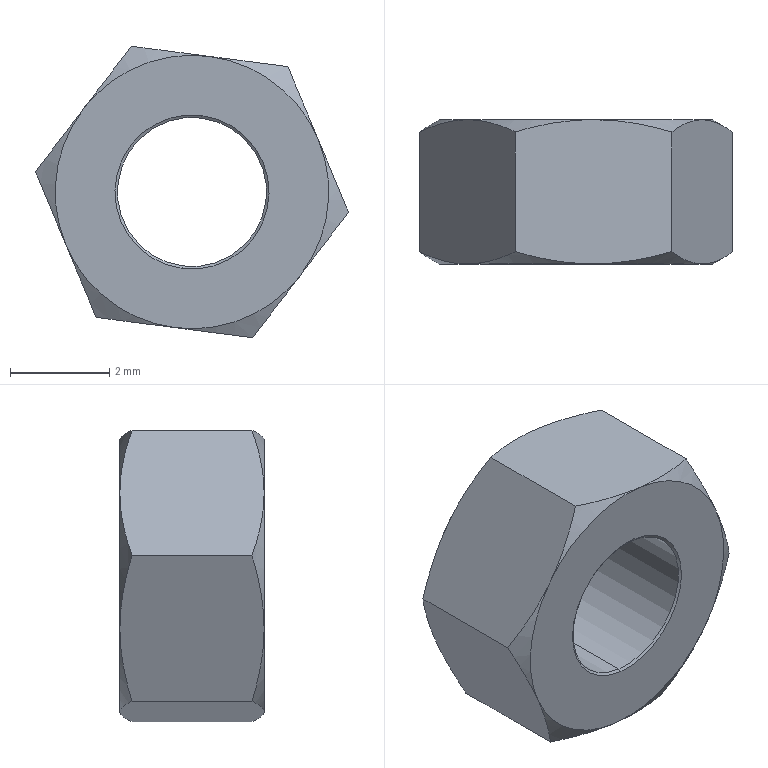Component | SolidWorks | hex nut style 2_am_pkg-1 | 1 solid | 28 faces | box 6.3 x 2.9 x 5.86 mm | volume 55 mm3 | cone 16 | plane 8 | cylinder 4 | commonest cylinder face diameters 3.1 x2 3 x2
STEP:
#1=COLOUR_RGB('',0.7922,0.8196,0.9333);
#2=FILL_AREA_STYLE_COLOUR('',#1);
#3=FILL_AREA_STYLE('',(#2));
#4=SURFACE_STYLE_FILL_AREA(#3);
#5=SURFACE_SIDE_STYLE('',(#4));
#6=SURFACE_STYLE_USAGE(.BOTH.,#5);
#7=PRESENTATION_STYLE_ASSIGNMENT((#6));
#8=CARTESIAN_POINT('',(-0.8987,-0.,1.164));
#9=VERTEX_POINT('',#8);
#10=CARTESIAN_POINT('',(-0.883,-0.,1.285));
#11=VERTEX_POINT('',#10);
#12=CARTESIAN_POINT('',(-0.8908,-0.,1.225));
#13=DIRECTION('',(0.,-1.,0.));
#14=DIRECTION('',(-0.1287,-0.,-0.9917));
#15=AXIS2_PLACEMENT_3D('',#12,#13,#14);
#16=CIRCLE('',#15,0.06102);
#17=EDGE_CURVE('',#9,#11,#16,.T.);
#18=ORIENTED_EDGE('',*,*,#17,.F.);
#19=CARTESIAN_POINT('',(-0.8987,-0.001,1.164));
#20=VERTEX_POINT('',#19);
#21=CARTESIAN_POINT('',(-0.8987,0.8716,1.164));
#22=DIRECTION('',(0.,-1.,0.));
#23=VECTOR('',#22,39.37);
#24=LINE('',#21,#23);
#25=EDGE_CURVE('',#9,#20,#24,.T.);
#26=ORIENTED_EDGE('',*,*,#25,.T.);
#27=CARTESIAN_POINT('',(-0.883,-0.001,1.285));
#28=VERTEX_POINT('',#27);
#29=CARTESIAN_POINT('',(-0.8908,-0.001,1.225));
#30=DIRECTION('',(0.,-1.,0.));
#31=DIRECTION('',(0.1287,0.,0.9917));
#32=AXIS2_PLACEMENT_3D('',#29,#30,#31);
#33=CIRCLE('',#32,0.06102);
#34=EDGE_CURVE('',#20,#28,#33,.T.);
#35=ORIENTED_EDGE('',*,*,#34,.T.);
#36=CARTESIAN_POINT('',(-0.883,0.8716,1.285));
#37=DIRECTION('',(0.,-1.,0.));
#38=VECTOR('',#37,39.37);
#39=LINE('',#36,#38);
#40=EDGE_CURVE('',#11,#28,#39,.T.);
#41=ORIENTED_EDGE('',*,*,#40,.F.);
#42=EDGE_LOOP('',(#18,#26,#35,#41));
#43=FACE_OUTER_BOUND('',#42,.T.);
#44=CARTESIAN_POINT('',(-0.8908,0.8716,1.225));
#45=DIRECTION('',(0.,-1.,0.));
#46=DIRECTION('',(0.1287,0.,0.9917));
#47=AXIS2_PLACEMENT_3D('',#44,#45,#46);
#48=CYLINDRICAL_SURFACE('',#47,0.06102);
#49=ADVANCED_FACE('',(#43),#48,.F.);
#50=CARTESIAN_POINT('',(-0.8984,-0.002378,1.166));
#51=VERTEX_POINT('',#50);
#52=CARTESIAN_POINT('',(-0.8832,-0.002378,1.283));
#53=VERTEX_POINT('',#52);
#54=CARTESIAN_POINT('',(-0.8908,-0.002378,1.225));
#55=DIRECTION('',(0.,-1.,0.));
#56=DIRECTION('',(-0.1287,-0.,-0.9917));
#57=AXIS2_PLACEMENT_3D('',#54,#55,#56);
#58=CIRCLE('',#57,0.05906);
#59=EDGE_CURVE('',#51,#53,#58,.T.);
#60=ORIENTED_EDGE('',*,*,#59,.T.);
#61=CARTESIAN_POINT('',(-0.883,-0.001,1.285));
#62=DIRECTION('',(0.1054,0.5736,0.8123));
#63=VECTOR('',#62,39.37);
#64=LINE('',#61,#63);
#65=EDGE_CURVE('',#53,#28,#64,.T.);
#66=ORIENTED_EDGE('',*,*,#65,.T.);
#67=ORIENTED_EDGE('',*,*,#34,.F.);
#68=CARTESIAN_POINT('',(-0.8987,-0.001,1.164));
#69=DIRECTION('',(-0.1054,0.5736,-0.8123));
#70=VECTOR('',#69,39.37);
#71=LINE('',#68,#70);
#72=EDGE_CURVE('',#51,#20,#71,.T.);
#73=ORIENTED_EDGE('',*,*,#72,.F.);
#74=EDGE_LOOP('',(#60,#66,#67,#73));
#75=FACE_OUTER_BOUND('',#74,.T.);
#76=CARTESIAN_POINT('',(-0.8908,-0.001,1.225));
#77=DIRECTION('',(-0.,1.,-0.));
#78=DIRECTION('',(-0.1287,-0.,-0.9917));
#79=AXIS2_PLACEMENT_3D('',#76,#77,#78);
#80=CONICAL_SURFACE('',#79,0.06102,0.9599);
#81=ADVANCED_FACE('',(#75),#80,.F.);
#82=CARTESIAN_POINT('',(-0.8832,-0.1128,1.283));
#83=VERTEX_POINT('',#82);
#84=CARTESIAN_POINT('',(-0.8984,-0.1128,1.166));
#85=VERTEX_POINT('',#84);
#86=CARTESIAN_POINT('',(-0.8908,-0.1128,1.225));
#87=DIRECTION('',(-0.,1.,-0.));
#88=DIRECTION('',(0.1287,0.,0.9917));
#89=AXIS2_PLACEMENT_3D('',#86,#87,#88);
#90=CIRCLE('',#89,0.05906);
#91=EDGE_CURVE('',#83,#85,#90,.T.);
#92=ORIENTED_EDGE('',*,*,#91,.T.);
#93=CARTESIAN_POINT('',(-0.8987,-0.1142,1.164));
#94=VERTEX_POINT('',#93);
#95=CARTESIAN_POINT('',(-0.8984,-0.1127,1.167));
#96=DIRECTION('',(-0.1054,-0.5736,-0.8123));
#97=VECTOR('',#96,39.37);
#98=LINE('',#95,#97);
#99=EDGE_CURVE('',#85,#94,#98,.T.);
#100=ORIENTED_EDGE('',*,*,#99,.T.);
#101=CARTESIAN_POINT('',(-0.883,-0.1142,1.285));
#102=VERTEX_POINT('',#101);
#103=CARTESIAN_POINT('',(-0.8908,-0.1142,1.225));
#104=DIRECTION('',(0.,-1.,0.));
#105=DIRECTION('',(0.1287,0.,0.9917));
#106=AXIS2_PLACEMENT_3D('',#103,#104,#105);
#107=CIRCLE('',#106,0.06102);
#108=EDGE_CURVE('',#94,#102,#107,.T.);
#109=ORIENTED_EDGE('',*,*,#108,.T.);
#110=CARTESIAN_POINT('',(-0.8833,-0.1127,1.283));
#111=DIRECTION('',(0.1054,-0.5736,0.8123));
#112=VECTOR('',#111,39.37);
#113=LINE('',#110,#112);
#114=EDGE_CURVE('',#83,#102,#113,.T.);
#115=ORIENTED_EDGE('',*,*,#114,.F.);
#116=EDGE_LOOP('',(#92,#100,#109,#115));
#117=FACE_OUTER_BOUND('',#116,.T.);
#118=CARTESIAN_POINT('',(-0.8908,-0.1127,1.225));
#119=DIRECTION('',(0.,-1.,0.));
#120=DIRECTION('',(0.1287,0.,0.9917));
#121=AXIS2_PLACEMENT_3D('',#118,#119,#120);
#122=CONICAL_SURFACE('',#121,0.05886,0.9599);
#123=ADVANCED_FACE('',(#117),#122,.F.);
#124=ORIENTED_EDGE('',*,*,#59,.F.);
#125=CARTESIAN_POINT('',(-0.8984,-0.,1.166));
#126=DIRECTION('',(0.,-1.,0.));
#127=VECTOR('',#126,39.37);
#128=LINE('',#125,#127);
#129=EDGE_CURVE('',#51,#85,#128,.T.);
#130=ORIENTED_EDGE('',*,*,#129,.T.);
#131=ORIENTED_EDGE('',*,*,#91,.F.);
#132=CARTESIAN_POINT('',(-0.8832,-0.,1.283));
#133=DIRECTION('',(0.,-1.,0.));
#134=VECTOR('',#133,39.37);
#135=LINE('',#132,#134);
#136=EDGE_CURVE('',#53,#83,#135,.T.);
#137=ORIENTED_EDGE('',*,*,#136,.F.);
#138=EDGE_LOOP('',(#124,#130,#131,#137));
#139=FACE_OUTER_BOUND('',#138,.T.);
#140=CARTESIAN_POINT('',(-0.8908,-0.,1.225));
#141=DIRECTION('',(0.,-1.,0.));
#142=DIRECTION('',(0.1287,0.,0.9917));
#143=AXIS2_PLACEMENT_3D('',#140,#141,#142);
#144=CYLINDRICAL_SURFACE('',#143,0.05906);
#145=ADVANCED_FACE('',(#139),#144,.F.);
#146=ORIENTED_EDGE('',*,*,#129,.F.);
#147=CARTESIAN_POINT('',(-0.8908,-0.002378,1.225));
#148=DIRECTION('',(0.,-1.,0.));
#149=DIRECTION('',(-0.1287,-0.,-0.9917));
#150=AXIS2_PLACEMENT_3D('',#147,#148,#149);
#151=CIRCLE('',#150,0.05906);
#152=EDGE_CURVE('',#53,#51,#151,.T.);
#153=ORIENTED_EDGE('',*,*,#152,.F.);
#154=ORIENTED_EDGE('',*,*,#136,.T.);
#155=CARTESIAN_POINT('',(-0.8908,-0.1128,1.225));
#156=DIRECTION('',(-0.,1.,-0.));
#157=DIRECTION('',(0.1287,0.,0.9917));
#158=AXIS2_PLACEMENT_3D('',#155,#156,#157);
#159=CIRCLE('',#158,0.05906);
#160=EDGE_CURVE('',#85,#83,#159,.T.);
#161=ORIENTED_EDGE('',*,*,#160,.F.);
#162=EDGE_LOOP('',(#146,#153,#154,#161));
#163=FACE_OUTER_BOUND('',#162,.T.);
#164=CARTESIAN_POINT('',(-0.8908,-0.,1.225));
#165=DIRECTION('',(0.,-1.,0.));
#166=DIRECTION('',(0.1287,0.,0.9917));
#167=AXIS2_PLACEMENT_3D('',#164,#165,#166);
#168=CYLINDRICAL_SURFACE('',#167,0.05906);
#169=ADVANCED_FACE('',(#163),#168,.F.);
#170=CARTESIAN_POINT('',(-0.9668,-0.00967,1.126));
#171=VERTEX_POINT('',#170);
#172=CARTESIAN_POINT('',(-0.9668,-0.1045,1.126));
#173=VERTEX_POINT('',#172);
#174=CARTESIAN_POINT('',(-0.9668,-0.,1.126));
#175=DIRECTION('',(0.,-1.,0.));
#176=VECTOR('',#175,39.37);
#177=LINE('',#174,#176);
#178=EDGE_CURVE('',#171,#173,#177,.T.);
#179=ORIENTED_EDGE('',*,*,#178,.T.);
#180=CARTESIAN_POINT('',(-0.9908,-0.1142,1.183));
#181=VERTEX_POINT('',#180);
#182=CARTESIAN_POINT('',(-0.9668,-0.1045,1.126));
#183=CARTESIAN_POINT('',(-0.9746,-0.1104,1.144));
#184=CARTESIAN_POINT('',(-0.9826,-0.1142,1.164));
#185=CARTESIAN_POINT('',(-0.9908,-0.1142,1.183));
#186=B_SPLINE_CURVE_WITH_KNOTS('',3,(#182,#183,#184,#185),.UNSPECIFIED.,.F.,.F.,(4,4),(0.00000024,0.001607),.UNSPECIFIED.);
#187=EDGE_CURVE('',#173,#181,#186,.T.);
#188=ORIENTED_EDGE('',*,*,#187,.T.);
#189=CARTESIAN_POINT('',(-1.015,-0.1045,1.241));
#190=VERTEX_POINT('',#189);
#191=CARTESIAN_POINT('',(-0.9908,-0.1142,1.183));
#192=CARTESIAN_POINT('',(-0.9949,-0.1142,1.193));
#193=CARTESIAN_POINT('',(-0.9989,-0.1132,1.203));
#194=CARTESIAN_POINT('',(-1.007,-0.1099,1.222));
#195=CARTESIAN_POINT('',(-1.011,-0.1074,1.232));
#196=CARTESIAN_POINT('',(-1.015,-0.1045,1.241));
#197=B_SPLINE_CURVE_WITH_KNOTS('',3,(#191,#192,#193,#194,#195,#196),.UNSPECIFIED.,.F.,.F.,(4,2,4),(0.001607,0.002407,0.003207),.UNSPECIFIED.);
#198=EDGE_CURVE('',#181,#190,#197,.T.);
#199=ORIENTED_EDGE('',*,*,#198,.T.);
#200=CARTESIAN_POINT('',(-1.015,-0.00967,1.241));
#201=VERTEX_POINT('',#200);
#202=CARTESIAN_POINT('',(-1.015,-0.,1.241));
#203=DIRECTION('',(0.,-1.,0.));
#204=VECTOR('',#203,39.37);
#205=LINE('',#202,#204);
#206=EDGE_CURVE('',#201,#190,#205,.T.);
#207=ORIENTED_EDGE('',*,*,#206,.F.);
#208=CARTESIAN_POINT('',(-0.9908,-0.,1.183));
#209=VERTEX_POINT('',#208);
#210=CARTESIAN_POINT('',(-0.9908,-0.,1.183));
#211=CARTESIAN_POINT('',(-0.9949,0.,1.193));
#212=CARTESIAN_POINT('',(-0.9989,-0.000926,1.203));
#213=CARTESIAN_POINT('',(-1.007,-0.004295,1.222));
#214=CARTESIAN_POINT('',(-1.011,-0.006726,1.232));
#215=CARTESIAN_POINT('',(-1.015,-0.00967,1.241));
#216=B_SPLINE_CURVE_WITH_KNOTS('',3,(#210,#211,#212,#213,#214,#215),.UNSPECIFIED.,.F.,.F.,(4,2,4),(0.001607,0.002407,0.003207),.UNSPECIFIED.);
#217=EDGE_CURVE('',#209,#201,#216,.T.);
#218=ORIENTED_EDGE('',*,*,#217,.F.);
#219=CARTESIAN_POINT('',(-0.9668,-0.00967,1.126));
#220=CARTESIAN_POINT('',(-0.9746,-0.003766,1.144));
#221=CARTESIAN_POINT('',(-0.9826,0.,1.164));
#222=CARTESIAN_POINT('',(-0.9908,-0.,1.183));
#223=B_SPLINE_CURVE_WITH_KNOTS('',3,(#219,#220,#221,#222),.UNSPECIFIED.,.F.,.F.,(4,4),(0.00000024,0.001607),.UNSPECIFIED.);
#224=EDGE_CURVE('',#171,#209,#223,.T.);
#225=ORIENTED_EDGE('',*,*,#224,.F.);
#226=EDGE_LOOP('',(#179,#188,#199,#207,#218,#225));
#227=FACE_OUTER_BOUND('',#226,.T.);
#228=CARTESIAN_POINT('',(-1.015,-0.,1.241));
#229=DIRECTION('',(-0.9232,-0.,-0.3844));
#230=DIRECTION('',(0.3844,-0.,-0.9232));
#231=AXIS2_PLACEMENT_3D('',#228,#229,#230);
#232=PLANE('',#231);
#233=ADVANCED_FACE('',(#227),#232,.T.);
#234=ORIENTED_EDGE('',*,*,#206,.T.);
#235=CARTESIAN_POINT('',(-0.9769,-0.1142,1.291));
#236=VERTEX_POINT('',#235);
#237=CARTESIAN_POINT('',(-1.015,-0.1045,1.241));
#238=CARTESIAN_POINT('',(-1.002,-0.1104,1.257));
#239=CARTESIAN_POINT('',(-0.9898,-0.1142,1.274));
#240=CARTESIAN_POINT('',(-0.9769,-0.1142,1.291));
#241=B_SPLINE_CURVE_WITH_KNOTS('',3,(#237,#238,#239,#240),.UNSPECIFIED.,.F.,.F.,(4,4),(0.00000024,0.001607),.UNSPECIFIED.);
#242=EDGE_CURVE('',#190,#236,#241,.T.);
#243=ORIENTED_EDGE('',*,*,#242,.T.);
#244=CARTESIAN_POINT('',(-0.9389,-0.1045,1.34));
#245=VERTEX_POINT('',#244);
#246=CARTESIAN_POINT('',(-0.9769,-0.1142,1.291));
#247=CARTESIAN_POINT('',(-0.9704,-0.1142,1.299));
#248=CARTESIAN_POINT('',(-0.964,-0.1132,1.308));
#249=CARTESIAN_POINT('',(-0.9513,-0.1099,1.324));
#250=CARTESIAN_POINT('',(-0.9451,-0.1074,1.332));
#251=CARTESIAN_POINT('',(-0.9389,-0.1045,1.34));
#252=B_SPLINE_CURVE_WITH_KNOTS('',3,(#246,#247,#248,#249,#250,#251),.UNSPECIFIED.,.F.,.F.,(4,2,4),(0.001607,0.002407,0.003207),.UNSPECIFIED.);
#253=EDGE_CURVE('',#236,#245,#252,.T.);
#254=ORIENTED_EDGE('',*,*,#253,.T.);
#255=CARTESIAN_POINT('',(-0.9389,-0.00967,1.34));
#256=VERTEX_POINT('',#255);
#257=CARTESIAN_POINT('',(-0.9389,-0.,1.34));
#258=DIRECTION('',(0.,-1.,0.));
#259=VECTOR('',#258,39.37);
#260=LINE('',#257,#259);
#261=EDGE_CURVE('',#256,#245,#260,.T.);
#262=ORIENTED_EDGE('',*,*,#261,.F.);
#263=CARTESIAN_POINT('',(-0.9769,-0.,1.291));
#264=VERTEX_POINT('',#263);
#265=CARTESIAN_POINT('',(-0.9769,-0.,1.291));
#266=CARTESIAN_POINT('',(-0.9704,0.,1.299));
#267=CARTESIAN_POINT('',(-0.964,-0.000926,1.308));
#268=CARTESIAN_POINT('',(-0.9513,-0.004295,1.324));
#269=CARTESIAN_POINT('',(-0.9451,-0.006726,1.332));
#270=CARTESIAN_POINT('',(-0.9389,-0.00967,1.34));
#271=B_SPLINE_CURVE_WITH_KNOTS('',3,(#265,#266,#267,#268,#269,#270),.UNSPECIFIED.,.F.,.F.,(4,2,4),(0.001607,0.002407,0.003207),.UNSPECIFIED.);
#272=EDGE_CURVE('',#264,#256,#271,.T.);
#273=ORIENTED_EDGE('',*,*,#272,.F.);
#274=CARTESIAN_POINT('',(-1.015,-0.00967,1.241));
#275=CARTESIAN_POINT('',(-1.002,-0.003766,1.257));
#276=CARTESIAN_POINT('',(-0.9898,0.,1.274));
#277=CARTESIAN_POINT('',(-0.9769,-0.,1.291));
#278=B_SPLINE_CURVE_WITH_KNOTS('',3,(#274,#275,#276,#277),.UNSPECIFIED.,.F.,.F.,(4,4),(0.00000024,0.001607),.UNSPECIFIED.);
#279=EDGE_CURVE('',#201,#264,#278,.T.);
#280=ORIENTED_EDGE('',*,*,#279,.F.);
#281=EDGE_LOOP('',(#234,#243,#254,#262,#273,#280));
#282=FACE_OUTER_BOUND('',#281,.T.);
#283=CARTESIAN_POINT('',(-0.9389,-0.,1.34));
#284=DIRECTION('',(-0.7945,-0.,0.6073));
#285=DIRECTION('',(-0.6073,-0.,-0.7945));
#286=AXIS2_PLACEMENT_3D('',#283,#284,#285);
#287=PLANE('',#286);
#288=ADVANCED_FACE('',(#282),#287,.T.);
#289=CARTESIAN_POINT('',(-0.8149,-0.1045,1.324));
#290=VERTEX_POINT('',#289);
#291=CARTESIAN_POINT('',(-0.8769,-0.1142,1.332));
#292=VERTEX_POINT('',#291);
#293=CARTESIAN_POINT('',(-0.8149,-0.1045,1.324));
#294=CARTESIAN_POINT('',(-0.825,-0.1074,1.326));
#295=CARTESIAN_POINT('',(-0.8353,-0.1099,1.327));
#296=CARTESIAN_POINT('',(-0.856,-0.1133,1.33));
#297=CARTESIAN_POINT('',(-0.8664,-0.1142,1.331));
#298=CARTESIAN_POINT('',(-0.8769,-0.1142,1.332));
#299=B_SPLINE_CURVE_WITH_KNOTS('',3,(#293,#294,#295,#296,#297,#298),.UNSPECIFIED.,.F.,.F.,(4,2,4),(0.002833,0.003636,0.004439),.UNSPECIFIED.);
#300=EDGE_CURVE('',#290,#292,#299,.T.);
#301=ORIENTED_EDGE('',*,*,#300,.F.);
#302=CARTESIAN_POINT('',(-0.8149,-0.00967,1.324));
#303=VERTEX_POINT('',#302);
#304=CARTESIAN_POINT('',(-0.8149,0.,1.324));
#305=DIRECTION('',(0.,-1.,0.));
#306=VECTOR('',#305,39.37);
#307=LINE('',#304,#306);
#308=EDGE_CURVE('',#303,#290,#307,.T.);
#309=ORIENTED_EDGE('',*,*,#308,.F.);
#310=CARTESIAN_POINT('',(-0.8769,-0.,1.332));
#311=VERTEX_POINT('',#310);
#312=CARTESIAN_POINT('',(-0.8149,-0.00967,1.324));
#313=CARTESIAN_POINT('',(-0.825,-0.006735,1.326));
#314=CARTESIAN_POINT('',(-0.8353,-0.004274,1.327));
#315=CARTESIAN_POINT('',(-0.856,-0.0009079,1.33));
#316=CARTESIAN_POINT('',(-0.8664,0.,1.331));
#317=CARTESIAN_POINT('',(-0.8769,-0.,1.332));
#318=B_SPLINE_CURVE_WITH_KNOTS('',3,(#312,#313,#314,#315,#316,#317),.UNSPECIFIED.,.F.,.F.,(4,2,4),(0.002833,0.003636,0.004439),.UNSPECIFIED.);
#319=EDGE_CURVE('',#303,#311,#318,.T.);
#320=ORIENTED_EDGE('',*,*,#319,.T.);
#321=CARTESIAN_POINT('',(-0.8769,-0.,1.332));
#322=CARTESIAN_POINT('',(-0.8874,0.,1.334));
#323=CARTESIAN_POINT('',(-0.898,-0.0009331,1.335));
#324=CARTESIAN_POINT('',(-0.9187,-0.004322,1.338));
#325=CARTESIAN_POINT('',(-0.9289,-0.006752,1.339));
#326=CARTESIAN_POINT('',(-0.9389,-0.00967,1.34));
#327=B_SPLINE_CURVE_WITH_KNOTS('',3,(#321,#322,#323,#324,#325,#326),.UNSPECIFIED.,.F.,.F.,(4,2,4),(0.004439,0.005242,0.006046),.UNSPECIFIED.);
#328=EDGE_CURVE('',#311,#256,#327,.T.);
#329=ORIENTED_EDGE('',*,*,#328,.T.);
#330=ORIENTED_EDGE('',*,*,#261,.T.);
#331=CARTESIAN_POINT('',(-0.8769,-0.1142,1.332));
#332=CARTESIAN_POINT('',(-0.8874,-0.1142,1.334));
#333=CARTESIAN_POINT('',(-0.898,-0.1132,1.335));
#334=CARTESIAN_POINT('',(-0.9187,-0.1099,1.338));
#335=CARTESIAN_POINT('',(-0.9289,-0.1074,1.339));
#336=CARTESIAN_POINT('',(-0.9389,-0.1045,1.34));
#337=B_SPLINE_CURVE_WITH_KNOTS('',3,(#331,#332,#333,#334,#335,#336),.UNSPECIFIED.,.F.,.F.,(4,2,4),(0.004439,0.005242,0.006046),.UNSPECIFIED.);
#338=EDGE_CURVE('',#292,#245,#337,.T.);
#339=ORIENTED_EDGE('',*,*,#338,.F.);
#340=EDGE_LOOP('',(#301,#309,#320,#329,#330,#339));
#341=FACE_OUTER_BOUND('',#340,.T.);
#342=CARTESIAN_POINT('',(-0.9389,-0.,1.34));
#343=DIRECTION('',(-0.1287,-0.,-0.9917));
#344=DIRECTION('',(0.,-1.,0.));
#345=AXIS2_PLACEMENT_3D('',#342,#343,#344);
#346=PLANE('',#345);
#347=ADVANCED_FACE('',(#341),#346,.F.);
#348=ORIENTED_EDGE('',*,*,#308,.T.);
#349=CARTESIAN_POINT('',(-0.7909,-0.1142,1.267));
#350=VERTEX_POINT('',#349);
#351=CARTESIAN_POINT('',(-0.8149,-0.1045,1.324));
#352=CARTESIAN_POINT('',(-0.8071,-0.1104,1.305));
#353=CARTESIAN_POINT('',(-0.7991,-0.1142,1.286));
#354=CARTESIAN_POINT('',(-0.7909,-0.1142,1.267));
#355=B_SPLINE_CURVE_WITH_KNOTS('',3,(#351,#352,#353,#354),.UNSPECIFIED.,.F.,.F.,(4,4),(0.00000024,0.001607),.UNSPECIFIED.);
#356=EDGE_CURVE('',#290,#350,#355,.T.);
#357=ORIENTED_EDGE('',*,*,#356,.T.);
#358=CARTESIAN_POINT('',(-0.7669,-0.1045,1.209));
#359=VERTEX_POINT('',#358);
#360=CARTESIAN_POINT('',(-0.7909,-0.1142,1.267));
#361=CARTESIAN_POINT('',(-0.7868,-0.1142,1.257));
#362=CARTESIAN_POINT('',(-0.7827,-0.1132,1.247));
#363=CARTESIAN_POINT('',(-0.7747,-0.1099,1.228));
#364=CARTESIAN_POINT('',(-0.7708,-0.1074,1.218));
#365=CARTESIAN_POINT('',(-0.7669,-0.1045,1.209));
#366=B_SPLINE_CURVE_WITH_KNOTS('',3,(#360,#361,#362,#363,#364,#365),.UNSPECIFIED.,.F.,.F.,(4,2,4),(0.001607,0.002407,0.003207),.UNSPECIFIED.);
#367=EDGE_CURVE('',#350,#359,#366,.T.);
#368=ORIENTED_EDGE('',*,*,#367,.T.);
#369=CARTESIAN_POINT('',(-0.7669,-0.00967,1.209));
#370=VERTEX_POINT('',#369);
#371=CARTESIAN_POINT('',(-0.7669,0.,1.209));
#372=DIRECTION('',(0.,-1.,0.));
#373=VECTOR('',#372,39.37);
#374=LINE('',#371,#373);
#375=EDGE_CURVE('',#370,#359,#374,.T.);
#376=ORIENTED_EDGE('',*,*,#375,.F.);
#377=CARTESIAN_POINT('',(-0.7909,0.,1.267));
#378=VERTEX_POINT('',#377);
#379=CARTESIAN_POINT('',(-0.7909,0.,1.267));
#380=CARTESIAN_POINT('',(-0.7868,-0.,1.257));
#381=CARTESIAN_POINT('',(-0.7827,-0.000926,1.247));
#382=CARTESIAN_POINT('',(-0.7747,-0.004295,1.228));
#383=CARTESIAN_POINT('',(-0.7708,-0.006726,1.218));
#384=CARTESIAN_POINT('',(-0.7669,-0.00967,1.209));
#385=B_SPLINE_CURVE_WITH_KNOTS('',3,(#379,#380,#381,#382,#383,#384),.UNSPECIFIED.,.F.,.F.,(4,2,4),(0.001607,0.002407,0.003207),.UNSPECIFIED.);
#386=EDGE_CURVE('',#378,#370,#385,.T.);
#387=ORIENTED_EDGE('',*,*,#386,.F.);
#388=CARTESIAN_POINT('',(-0.8149,-0.00967,1.324));
#389=CARTESIAN_POINT('',(-0.8071,-0.003766,1.305));
#390=CARTESIAN_POINT('',(-0.7991,-0.,1.286));
#391=CARTESIAN_POINT('',(-0.7909,0.,1.267));
#392=B_SPLINE_CURVE_WITH_KNOTS('',3,(#388,#389,#390,#391),.UNSPECIFIED.,.F.,.F.,(4,4),(0.00000024,0.001607),.UNSPECIFIED.);
#393=EDGE_CURVE('',#303,#378,#392,.T.);
#394=ORIENTED_EDGE('',*,*,#393,.F.);
#395=EDGE_LOOP('',(#348,#357,#368,#376,#387,#394));
#396=FACE_OUTER_BOUND('',#395,.T.);
#397=CARTESIAN_POINT('',(-0.7669,0.,1.209));
#398=DIRECTION('',(0.9232,0.,0.3844));
#399=DIRECTION('',(-0.3844,0.,0.9232));
#400=AXIS2_PLACEMENT_3D('',#397,#398,#399);
#401=PLANE('',#400);
#402=ADVANCED_FACE('',(#396),#401,.T.);
#403=ORIENTED_EDGE('',*,*,#375,.T.);
#404=CARTESIAN_POINT('',(-0.8048,-0.1142,1.159));
#405=VERTEX_POINT('',#404);
#406=CARTESIAN_POINT('',(-0.7669,-0.1045,1.209));
#407=CARTESIAN_POINT('',(-0.7793,-0.1104,1.193));
#408=CARTESIAN_POINT('',(-0.7919,-0.1142,1.176));
#409=CARTESIAN_POINT('',(-0.8048,-0.1142,1.159));
#410=B_SPLINE_CURVE_WITH_KNOTS('',3,(#406,#407,#408,#409),.UNSPECIFIED.,.F.,.F.,(4,4),(0.00000024,0.001607),.UNSPECIFIED.);
#411=EDGE_CURVE('',#359,#405,#410,.T.);
#412=ORIENTED_EDGE('',*,*,#411,.T.);
#413=CARTESIAN_POINT('',(-0.8428,-0.1045,1.109));
#414=VERTEX_POINT('',#413);
#415=CARTESIAN_POINT('',(-0.8048,-0.1142,1.159));
#416=CARTESIAN_POINT('',(-0.8113,-0.1142,1.151));
#417=CARTESIAN_POINT('',(-0.8177,-0.1132,1.142));
#418=CARTESIAN_POINT('',(-0.8303,-0.1099,1.126));
#419=CARTESIAN_POINT('',(-0.8366,-0.1074,1.118));
#420=CARTESIAN_POINT('',(-0.8428,-0.1045,1.109));
#421=B_SPLINE_CURVE_WITH_KNOTS('',3,(#415,#416,#417,#418,#419,#420),.UNSPECIFIED.,.F.,.F.,(4,2,4),(0.001607,0.002407,0.003207),.UNSPECIFIED.);
#422=EDGE_CURVE('',#405,#414,#421,.T.);
#423=ORIENTED_EDGE('',*,*,#422,.T.);
#424=CARTESIAN_POINT('',(-0.8428,-0.00967,1.109));
#425=VERTEX_POINT('',#424);
#426=CARTESIAN_POINT('',(-0.8428,-0.,1.109));
#427=DIRECTION('',(0.,-1.,0.));
#428=VECTOR('',#427,39.37);
#429=LINE('',#426,#428);
#430=EDGE_CURVE('',#425,#414,#429,.T.);
#431=ORIENTED_EDGE('',*,*,#430,.F.);
#432=CARTESIAN_POINT('',(-0.8048,-0.,1.159));
#433=VERTEX_POINT('',#432);
#434=CARTESIAN_POINT('',(-0.8048,-0.,1.159));
#435=CARTESIAN_POINT('',(-0.8113,-0.,1.151));
#436=CARTESIAN_POINT('',(-0.8177,-0.000926,1.142));
#437=CARTESIAN_POINT('',(-0.8303,-0.004295,1.126));
#438=CARTESIAN_POINT('',(-0.8366,-0.006726,1.118));
#439=CARTESIAN_POINT('',(-0.8428,-0.00967,1.109));
#440=B_SPLINE_CURVE_WITH_KNOTS('',3,(#434,#435,#436,#437,#438,#439),.UNSPECIFIED.,.F.,.F.,(4,2,4),(0.001607,0.002407,0.003207),.UNSPECIFIED.);
#441=EDGE_CURVE('',#433,#425,#440,.T.);
#442=ORIENTED_EDGE('',*,*,#441,.F.);
#443=CARTESIAN_POINT('',(-0.7669,-0.00967,1.209));
#444=CARTESIAN_POINT('',(-0.7793,-0.003766,1.193));
#445=CARTESIAN_POINT('',(-0.7919,-0.,1.176));
#446=CARTESIAN_POINT('',(-0.8048,-0.,1.159));
#447=B_SPLINE_CURVE_WITH_KNOTS('',3,(#443,#444,#445,#446),.UNSPECIFIED.,.F.,.F.,(4,4),(0.00000024,0.001607),.UNSPECIFIED.);
#448=EDGE_CURVE('',#370,#433,#447,.T.);
#449=ORIENTED_EDGE('',*,*,#448,.F.);
#450=EDGE_LOOP('',(#403,#412,#423,#431,#442,#449));
#451=FACE_OUTER_BOUND('',#450,.T.);
#452=CARTESIAN_POINT('',(-0.8428,-0.,1.109));
#453=DIRECTION('',(0.7945,0.,-0.6073));
#454=DIRECTION('',(0.6073,0.,0.7945));
#455=AXIS2_PLACEMENT_3D('',#452,#453,#454);
#456=PLANE('',#455);
#457=ADVANCED_FACE('',(#451),#456,.T.);
#458=ORIENTED_EDGE('',*,*,#430,.T.);
#459=CARTESIAN_POINT('',(-0.9048,-0.1142,1.118));
#460=VERTEX_POINT('',#459);
#461=CARTESIAN_POINT('',(-0.8428,-0.1045,1.109));
#462=CARTESIAN_POINT('',(-0.8529,-0.1074,1.111));
#463=CARTESIAN_POINT('',(-0.8632,-0.1099,1.112));
#464=CARTESIAN_POINT('',(-0.8839,-0.1133,1.115));
#465=CARTESIAN_POINT('',(-0.8943,-0.1142,1.116));
#466=CARTESIAN_POINT('',(-0.9048,-0.1142,1.118));
#467=B_SPLINE_CURVE_WITH_KNOTS('',3,(#461,#462,#463,#464,#465,#466),.UNSPECIFIED.,.F.,.F.,(4,2,4),(0.002833,0.003636,0.004439),.UNSPECIFIED.);
#468=EDGE_CURVE('',#414,#460,#467,.T.);
#469=ORIENTED_EDGE('',*,*,#468,.T.);
#470=CARTESIAN_POINT('',(-0.9048,-0.1142,1.118));
#471=CARTESIAN_POINT('',(-0.9153,-0.1142,1.119));
#472=CARTESIAN_POINT('',(-0.9259,-0.1132,1.12));
#473=CARTESIAN_POINT('',(-0.9466,-0.1099,1.123));
#474=CARTESIAN_POINT('',(-0.9567,-0.1074,1.124));
#475=CARTESIAN_POINT('',(-0.9668,-0.1045,1.126));
#476=B_SPLINE_CURVE_WITH_KNOTS('',3,(#470,#471,#472,#473,#474,#475),.UNSPECIFIED.,.F.,.F.,(4,2,4),(0.004439,0.005242,0.006046),.UNSPECIFIED.);
#477=EDGE_CURVE('',#460,#173,#476,.T.);
#478=ORIENTED_EDGE('',*,*,#477,.T.);
#479=ORIENTED_EDGE('',*,*,#178,.F.);
#480=CARTESIAN_POINT('',(-0.9048,-0.,1.118));
#481=VERTEX_POINT('',#480);
#482=CARTESIAN_POINT('',(-0.9048,-0.,1.118));
#483=CARTESIAN_POINT('',(-0.9153,0.,1.119));
#484=CARTESIAN_POINT('',(-0.9259,-0.0009331,1.12));
#485=CARTESIAN_POINT('',(-0.9466,-0.004322,1.123));
#486=CARTESIAN_POINT('',(-0.9567,-0.006752,1.124));
#487=CARTESIAN_POINT('',(-0.9668,-0.00967,1.126));
#488=B_SPLINE_CURVE_WITH_KNOTS('',3,(#482,#483,#484,#485,#486,#487),.UNSPECIFIED.,.F.,.F.,(4,2,4),(0.004439,0.005242,0.006046),.UNSPECIFIED.);
#489=EDGE_CURVE('',#481,#171,#488,.T.);
#490=ORIENTED_EDGE('',*,*,#489,.F.);
#491=CARTESIAN_POINT('',(-0.8428,-0.00967,1.109));
#492=CARTESIAN_POINT('',(-0.8529,-0.006735,1.111));
#493=CARTESIAN_POINT('',(-0.8632,-0.004274,1.112));
#494=CARTESIAN_POINT('',(-0.8839,-0.0009079,1.115));
#495=CARTESIAN_POINT('',(-0.8943,0.,1.116));
#496=CARTESIAN_POINT('',(-0.9048,-0.,1.118));
#497=B_SPLINE_CURVE_WITH_KNOTS('',3,(#491,#492,#493,#494,#495,#496),.UNSPECIFIED.,.F.,.F.,(4,2,4),(0.002833,0.003636,0.004439),.UNSPECIFIED.);
#498=EDGE_CURVE('',#425,#481,#497,.T.);
#499=ORIENTED_EDGE('',*,*,#498,.F.);
#500=EDGE_LOOP('',(#458,#469,#478,#479,#490,#499));
#501=FACE_OUTER_BOUND('',#500,.T.);
#502=CARTESIAN_POINT('',(-0.9668,-0.,1.126));
#503=DIRECTION('',(-0.1287,-0.,-0.9917));
#504=DIRECTION('',(0.,-1.,0.));
#505=AXIS2_PLACEMENT_3D('',#502,#503,#504);
#506=PLANE('',#505);
#507=ADVANCED_FACE('',(#501),#506,.T.);
#508=CARTESIAN_POINT('',(-0.8908,-0.1142,1.225));
#509=DIRECTION('',(0.,-1.,0.));
#510=DIRECTION('',(0.1287,0.,0.9917));
#511=AXIS2_PLACEMENT_3D('',#508,#509,#510);
#512=CIRCLE('',#511,0.06102);
#513=EDGE_CURVE('',#102,#94,#512,.T.);
#514=ORIENTED_EDGE('',*,*,#513,.F.);
#515=ORIENTED_EDGE('',*,*,#108,.F.);
#516=EDGE_LOOP('',(#514,#515));
#517=FACE_BOUND('',#516,.T.);
#518=CARTESIAN_POINT('',(-0.8908,-0.1142,1.225));
#519=DIRECTION('',(-0.,1.,-0.));
#520=DIRECTION('',(-0.1287,0.,-0.9917));
#521=AXIS2_PLACEMENT_3D('',#518,#519,#520);
#522=CIRCLE('',#521,0.1083);
#523=EDGE_CURVE('',#460,#181,#522,.T.);
#524=ORIENTED_EDGE('',*,*,#523,.F.);
#525=CARTESIAN_POINT('',(-0.8908,-0.1142,1.225));
#526=DIRECTION('',(-0.,1.,-0.));
#527=DIRECTION('',(-0.1287,0.,-0.9917));
#528=AXIS2_PLACEMENT_3D('',#525,#526,#527);
#529=CIRCLE('',#528,0.1083);
#530=EDGE_CURVE('',#405,#460,#529,.T.);
#531=ORIENTED_EDGE('',*,*,#530,.F.);
#532=CARTESIAN_POINT('',(-0.8908,-0.1142,1.225));
#533=DIRECTION('',(-0.,1.,-0.));
#534=DIRECTION('',(-0.1287,0.,-0.9917));
#535=AXIS2_PLACEMENT_3D('',#532,#533,#534);
#536=CIRCLE('',#535,0.1083);
#537=EDGE_CURVE('',#350,#405,#536,.T.);
#538=ORIENTED_EDGE('',*,*,#537,.F.);
#539=CARTESIAN_POINT('',(-0.8908,-0.1142,1.225));
#540=DIRECTION('',(-0.,1.,-0.));
#541=DIRECTION('',(-0.1287,0.,-0.9917));
#542=AXIS2_PLACEMENT_3D('',#539,#540,#541);
#543=CIRCLE('',#542,0.1083);
#544=EDGE_CURVE('',#292,#350,#543,.T.);
#545=ORIENTED_EDGE('',*,*,#544,.F.);
#546=CARTESIAN_POINT('',(-0.8908,-0.1142,1.225));
#547=DIRECTION('',(0.,-1.,0.));
#548=DIRECTION('',(0.1287,0.,0.9917));
#549=AXIS2_PLACEMENT_3D('',#546,#547,#548);
#550=CIRCLE('',#549,0.1083);
#551=EDGE_CURVE('',#292,#236,#550,.T.);
#552=ORIENTED_EDGE('',*,*,#551,.T.);
#553=CARTESIAN_POINT('',(-0.8908,-0.1142,1.225));
#554=DIRECTION('',(-0.,1.,-0.));
#555=DIRECTION('',(-0.1287,0.,-0.9917));
#556=AXIS2_PLACEMENT_3D('',#553,#554,#555);
#557=CIRCLE('',#556,0.1083);
#558=EDGE_CURVE('',#181,#236,#557,.T.);
#559=ORIENTED_EDGE('',*,*,#558,.F.);
#560=EDGE_LOOP('',(#524,#531,#538,#545,#552,#559));
#561=FACE_OUTER_BOUND('',#560,.T.);
#562=CARTESIAN_POINT('',(-1.015,-0.1142,1.241));
#563=DIRECTION('',(-0.,1.,-0.));
#564=DIRECTION('',(-0.1287,-0.,-0.9917));
#565=AXIS2_PLACEMENT_3D('',#562,#563,#564);
#566=PLANE('',#565);
#567=ADVANCED_FACE('',(#517,#561),#566,.F.);
#568=CARTESIAN_POINT('',(-0.8908,-0.,1.225));
#569=DIRECTION('',(0.,-1.,0.));
#570=DIRECTION('',(-0.1287,-0.,-0.9917));
#571=AXIS2_PLACEMENT_3D('',#568,#569,#570);
#572=CIRCLE('',#571,0.06102);
#573=EDGE_CURVE('',#11,#9,#572,.T.);
#574=ORIENTED_EDGE('',*,*,#573,.T.);
#575=ORIENTED_EDGE('',*,*,#17,.T.);
#576=EDGE_LOOP('',(#574,#575));
#577=FACE_BOUND('',#576,.T.);
#578=CARTESIAN_POINT('',(-0.8908,-0.,1.225));
#579=DIRECTION('',(0.,-1.,0.));
#580=DIRECTION('',(-0.1287,-0.,-0.9917));
#581=AXIS2_PLACEMENT_3D('',#578,#579,#580);
#582=CIRCLE('',#581,0.1083);
#583=EDGE_CURVE('',#481,#433,#582,.T.);
#584=ORIENTED_EDGE('',*,*,#583,.F.);
#585=CARTESIAN_POINT('',(-0.8908,-0.,1.225));
#586=DIRECTION('',(0.,-1.,0.));
#587=DIRECTION('',(-0.1287,-0.,-0.9917));
#588=AXIS2_PLACEMENT_3D('',#585,#586,#587);
#589=CIRCLE('',#588,0.1083);
#590=EDGE_CURVE('',#209,#481,#589,.T.);
#591=ORIENTED_EDGE('',*,*,#590,.F.);
#592=CARTESIAN_POINT('',(-0.8908,-0.,1.225));
#593=DIRECTION('',(0.,-1.,0.));
#594=DIRECTION('',(-0.1287,-0.,-0.9917));
#595=AXIS2_PLACEMENT_3D('',#592,#593,#594);
#596=CIRCLE('',#595,0.1083);
#597=EDGE_CURVE('',#264,#209,#596,.T.);
#598=ORIENTED_EDGE('',*,*,#597,.F.);
#599=CARTESIAN_POINT('',(-0.8908,-0.,1.225));
#600=DIRECTION('',(0.,-1.,0.));
#601=DIRECTION('',(0.1287,0.,0.9917));
#602=AXIS2_PLACEMENT_3D('',#599,#600,#601);
#603=CIRCLE('',#602,0.1083);
#604=EDGE_CURVE('',#311,#264,#603,.T.);
#605=ORIENTED_EDGE('',*,*,#604,.F.);
#606=CARTESIAN_POINT('',(-0.8908,-0.,1.225));
#607=DIRECTION('',(0.,-1.,0.));
#608=DIRECTION('',(-0.1287,-0.,-0.9917));
#609=AXIS2_PLACEMENT_3D('',#606,#607,#608);
#610=CIRCLE('',#609,0.1083);
#611=EDGE_CURVE('',#378,#311,#610,.T.);
#612=ORIENTED_EDGE('',*,*,#611,.F.);
#613=CARTESIAN_POINT('',(-0.8908,-0.,1.225));
#614=DIRECTION('',(0.,-1.,0.));
#615=DIRECTION('',(-0.1287,-0.,-0.9917));
#616=AXIS2_PLACEMENT_3D('',#613,#614,#615);
#617=CIRCLE('',#616,0.1083);
#618=EDGE_CURVE('',#433,#378,#617,.T.);
#619=ORIENTED_EDGE('',*,*,#618,.F.);
#620=EDGE_LOOP('',(#584,#591,#598,#605,#612,#619));
#621=FACE_OUTER_BOUND('',#620,.T.);
#622=CARTESIAN_POINT('',(-1.015,-0.,1.241));
#623=DIRECTION('',(-0.,1.,-0.));
#624=DIRECTION('',(-0.1287,-0.,-0.9917));
#625=AXIS2_PLACEMENT_3D('',#622,#623,#624);
#626=PLANE('',#625);
#627=ADVANCED_FACE('',(#577,#621),#626,.T.);
#628=ORIENTED_EDGE('',*,*,#224,.T.);
#629=ORIENTED_EDGE('',*,*,#590,.T.);
#630=ORIENTED_EDGE('',*,*,#489,.T.);
#631=EDGE_LOOP('',(#628,#629,#630));
#632=FACE_OUTER_BOUND('',#631,.T.);
#633=CARTESIAN_POINT('',(-0.8908,-0.,1.225));
#634=DIRECTION('',(0.,-1.,0.));
#635=DIRECTION('',(0.1287,0.,0.9917));
#636=AXIS2_PLACEMENT_3D('',#633,#634,#635);
#637=CONICAL_SURFACE('',#636,0.1083,1.047);
#638=ADVANCED_FACE('',(#632),#637,.T.);
#639=ORIENTED_EDGE('',*,*,#217,.T.);
#640=ORIENTED_EDGE('',*,*,#279,.T.);
#641=ORIENTED_EDGE('',*,*,#597,.T.);
#642=EDGE_LOOP('',(#639,#640,#641));
#643=FACE_OUTER_BOUND('',#642,.T.);
#644=CARTESIAN_POINT('',(-0.8908,-0.,1.225));
#645=DIRECTION('',(0.,-1.,0.));
#646=DIRECTION('',(0.1287,0.,0.9917));
#647=AXIS2_PLACEMENT_3D('',#644,#645,#646);
#648=CONICAL_SURFACE('',#647,0.1083,1.047);
#649=ADVANCED_FACE('',(#643),#648,.T.);
#650=ORIENTED_EDGE('',*,*,#272,.T.);
#651=ORIENTED_EDGE('',*,*,#328,.F.);
#652=ORIENTED_EDGE('',*,*,#604,.T.);
#653=EDGE_LOOP('',(#650,#651,#652));
#654=FACE_OUTER_BOUND('',#653,.T.);
#655=CARTESIAN_POINT('',(-0.8908,-0.,1.225));
#656=DIRECTION('',(0.,-1.,0.));
#657=DIRECTION('',(0.1287,0.,0.9917));
#658=AXIS2_PLACEMENT_3D('',#655,#656,#657);
#659=CONICAL_SURFACE('',#658,0.1083,1.047);
#660=ADVANCED_FACE('',(#654),#659,.T.);
#661=ORIENTED_EDGE('',*,*,#393,.T.);
#662=ORIENTED_EDGE('',*,*,#611,.T.);
#663=ORIENTED_EDGE('',*,*,#319,.F.);
#664=EDGE_LOOP('',(#661,#662,#663));
#665=FACE_OUTER_BOUND('',#664,.T.);
#666=CARTESIAN_POINT('',(-0.8908,-0.,1.225));
#667=DIRECTION('',(0.,-1.,0.));
#668=DIRECTION('',(0.1287,0.,0.9917));
#669=AXIS2_PLACEMENT_3D('',#666,#667,#668);
#670=CONICAL_SURFACE('',#669,0.1083,1.047);
#671=ADVANCED_FACE('',(#665),#670,.T.);
#672=ORIENTED_EDGE('',*,*,#386,.T.);
#673=ORIENTED_EDGE('',*,*,#448,.T.);
#674=ORIENTED_EDGE('',*,*,#618,.T.);
#675=EDGE_LOOP('',(#672,#673,#674));
#676=FACE_OUTER_BOUND('',#675,.T.);
#677=CARTESIAN_POINT('',(-0.8908,-0.,1.225));
#678=DIRECTION('',(0.,-1.,0.));
#679=DIRECTION('',(0.1287,0.,0.9917));
#680=AXIS2_PLACEMENT_3D('',#677,#678,#679);
#681=CONICAL_SURFACE('',#680,0.1083,1.047);
#682=ADVANCED_FACE('',(#676),#681,.T.);
#683=ORIENTED_EDGE('',*,*,#441,.T.);
#684=ORIENTED_EDGE('',*,*,#498,.T.);
#685=ORIENTED_EDGE('',*,*,#583,.T.);
#686=EDGE_LOOP('',(#683,#684,#685));
#687=FACE_OUTER_BOUND('',#686,.T.);
#688=CARTESIAN_POINT('',(-0.8908,-0.,1.225));
#689=DIRECTION('',(0.,-1.,0.));
#690=DIRECTION('',(0.1287,0.,0.9917));
#691=AXIS2_PLACEMENT_3D('',#688,#689,#690);
#692=CONICAL_SURFACE('',#691,0.1083,1.047);
#693=ADVANCED_FACE('',(#687),#692,.T.);
#694=ORIENTED_EDGE('',*,*,#530,.T.);
#695=ORIENTED_EDGE('',*,*,#468,.F.);
#696=ORIENTED_EDGE('',*,*,#422,.F.);
#697=EDGE_LOOP('',(#694,#695,#696));
#698=FACE_OUTER_BOUND('',#697,.T.);
#699=CARTESIAN_POINT('',(-0.8908,-0.1142,1.225));
#700=DIRECTION('',(-0.,1.,-0.));
#701=DIRECTION('',(-0.1287,0.,-0.9917));
#702=AXIS2_PLACEMENT_3D('',#699,#700,#701);
#703=CONICAL_SURFACE('',#702,0.1083,1.047);
#704=ADVANCED_FACE('',(#698),#703,.T.);
#705=ORIENTED_EDGE('',*,*,#537,.T.);
#706=ORIENTED_EDGE('',*,*,#411,.F.);
#707=ORIENTED_EDGE('',*,*,#367,.F.);
#708=EDGE_LOOP('',(#705,#706,#707));
#709=FACE_OUTER_BOUND('',#708,.T.);
#710=CARTESIAN_POINT('',(-0.8908,-0.1142,1.225));
#711=DIRECTION('',(-0.,1.,-0.));
#712=DIRECTION('',(-0.1287,0.,-0.9917));
#713=AXIS2_PLACEMENT_3D('',#710,#711,#712);
#714=CONICAL_SURFACE('',#713,0.1083,1.047);
#715=ADVANCED_FACE('',(#709),#714,.T.);
#716=ORIENTED_EDGE('',*,*,#300,.T.);
#717=ORIENTED_EDGE('',*,*,#544,.T.);
#718=ORIENTED_EDGE('',*,*,#356,.F.);
#719=EDGE_LOOP('',(#716,#717,#718));
#720=FACE_OUTER_BOUND('',#719,.T.);
#721=CARTESIAN_POINT('',(-0.8908,-0.1142,1.225));
#722=DIRECTION('',(-0.,1.,-0.));
#723=DIRECTION('',(-0.1287,0.,-0.9917));
#724=AXIS2_PLACEMENT_3D('',#721,#722,#723);
#725=CONICAL_SURFACE('',#724,0.1083,1.047);
#726=ADVANCED_FACE('',(#720),#725,.T.);
#727=ORIENTED_EDGE('',*,*,#551,.F.);
#728=ORIENTED_EDGE('',*,*,#338,.T.);
#729=ORIENTED_EDGE('',*,*,#253,.F.);
#730=EDGE_LOOP('',(#727,#728,#729));
#731=FACE_OUTER_BOUND('',#730,.T.);
#732=CARTESIAN_POINT('',(-0.8908,-0.1142,1.225));
#733=DIRECTION('',(-0.,1.,-0.));
#734=DIRECTION('',(-0.1287,0.,-0.9917));
#735=AXIS2_PLACEMENT_3D('',#732,#733,#734);
#736=CONICAL_SURFACE('',#735,0.1083,1.047);
#737=ADVANCED_FACE('',(#731),#736,.T.);
#738=ORIENTED_EDGE('',*,*,#558,.T.);
#739=ORIENTED_EDGE('',*,*,#242,.F.);
#740=ORIENTED_EDGE('',*,*,#198,.F.);
#741=EDGE_LOOP('',(#738,#739,#740));
#742=FACE_OUTER_BOUND('',#741,.T.);
#743=CARTESIAN_POINT('',(-0.8908,-0.1142,1.225));
#744=DIRECTION('',(-0.,1.,-0.));
#745=DIRECTION('',(-0.1287,0.,-0.9917));
#746=AXIS2_PLACEMENT_3D('',#743,#744,#745);
#747=CONICAL_SURFACE('',#746,0.1083,1.047);
#748=ADVANCED_FACE('',(#742),#747,.T.);
#749=ORIENTED_EDGE('',*,*,#477,.F.);
#750=ORIENTED_EDGE('',*,*,#523,.T.);
#751=ORIENTED_EDGE('',*,*,#187,.F.);
#752=EDGE_LOOP('',(#749,#750,#751));
#753=FACE_OUTER_BOUND('',#752,.T.);
#754=CARTESIAN_POINT('',(-0.8908,-0.1142,1.225));
#755=DIRECTION('',(-0.,1.,-0.));
#756=DIRECTION('',(-0.1287,0.,-0.9917));
#757=AXIS2_PLACEMENT_3D('',#754,#755,#756);
#758=CONICAL_SURFACE('',#757,0.1083,1.047);
#759=ADVANCED_FACE('',(#753),#758,.T.);
#760=ORIENTED_EDGE('',*,*,#99,.F.);
#761=ORIENTED_EDGE('',*,*,#160,.T.);
#762=ORIENTED_EDGE('',*,*,#114,.T.);
#763=ORIENTED_EDGE('',*,*,#513,.T.);
#764=EDGE_LOOP('',(#760,#761,#762,#763));
#765=FACE_OUTER_BOUND('',#764,.T.);
#766=CARTESIAN_POINT('',(-0.8908,-0.1127,1.225));
#767=DIRECTION('',(0.,-1.,0.));
#768=DIRECTION('',(0.1287,0.,0.9917));
#769=AXIS2_PLACEMENT_3D('',#766,#767,#768);
#770=CONICAL_SURFACE('',#769,0.05886,0.9599);
#771=ADVANCED_FACE('',(#765),#770,.F.);
#772=ORIENTED_EDGE('',*,*,#65,.F.);
#773=ORIENTED_EDGE('',*,*,#152,.T.);
#774=ORIENTED_EDGE('',*,*,#72,.T.);
#775=CARTESIAN_POINT('',(-0.8908,-0.001,1.225));
#776=DIRECTION('',(0.,-1.,0.));
#777=DIRECTION('',(0.1287,0.,0.9917));
#778=AXIS2_PLACEMENT_3D('',#775,#776,#777);
#779=CIRCLE('',#778,0.06102);
#780=EDGE_CURVE('',#28,#20,#779,.T.);
#781=ORIENTED_EDGE('',*,*,#780,.F.);
#782=EDGE_LOOP('',(#772,#773,#774,#781));
#783=FACE_OUTER_BOUND('',#782,.T.);
#784=CARTESIAN_POINT('',(-0.8908,-0.001,1.225));
#785=DIRECTION('',(-0.,1.,-0.));
#786=DIRECTION('',(-0.1287,-0.,-0.9917));
#787=AXIS2_PLACEMENT_3D('',#784,#785,#786);
#788=CONICAL_SURFACE('',#787,0.06102,0.9599);
#789=ADVANCED_FACE('',(#783),#788,.F.);
#790=ORIENTED_EDGE('',*,*,#25,.F.);
#791=ORIENTED_EDGE('',*,*,#573,.F.);
#792=ORIENTED_EDGE('',*,*,#40,.T.);
#793=ORIENTED_EDGE('',*,*,#780,.T.);
#794=EDGE_LOOP('',(#790,#791,#792,#793));
#795=FACE_OUTER_BOUND('',#794,.T.);
#796=CARTESIAN_POINT('',(-0.8908,0.8716,1.225));
#797=DIRECTION('',(0.,-1.,0.));
#798=DIRECTION('',(0.1287,0.,0.9917));
#799=AXIS2_PLACEMENT_3D('',#796,#797,#798);
#800=CYLINDRICAL_SURFACE('',#799,0.06102);
#801=ADVANCED_FACE('',(#795),#800,.F.);
#802=CLOSED_SHELL('',(#49,#81,#123,#145,#169,#233,#288,#347,#402,#457,#507,#567,#627,#638,#649,#660,#671,#682,#693,#704,#715,#726,#737,#748,#759,#771,#789,#801));
#803=MANIFOLD_SOLID_BREP('',#802);
#804=STYLED_ITEM('',(#7),#803);
#805=PRESENTATION_LAYER_ASSIGNMENT('','',(#804));
#806=(LENGTH_UNIT()NAMED_UNIT(*)SI_UNIT($,.METRE.));
#807=LENGTH_MEASURE_WITH_UNIT(LENGTH_MEASURE(0.0254),#806);
#808=DIMENSIONAL_EXPONENTS(1.,0.,0.,0.,0.,0.,0.);
#809=(CONVERSION_BASED_UNIT('',#807)LENGTH_UNIT()NAMED_UNIT(#808));
#810=UNCERTAINTY_MEASURE_WITH_UNIT(LENGTH_MEASURE(0.00001),#809,'','');
#811=(NAMED_UNIT(*)PLANE_ANGLE_UNIT()SI_UNIT($,.RADIAN.));
#812=(NAMED_UNIT(*)SI_UNIT($,.STERADIAN.)SOLID_ANGLE_UNIT());
#813=(GEOMETRIC_REPRESENTATION_CONTEXT(3)GLOBAL_UNCERTAINTY_ASSIGNED_CONTEXT((#810))GLOBAL_UNIT_ASSIGNED_CONTEXT((#809,#811,#812))REPRESENTATION_CONTEXT('',''));
#814=MECHANICAL_DESIGN_GEOMETRIC_PRESENTATION_REPRESENTATION('',(#804),#813);
#815=CARTESIAN_POINT('',(0.,0.,0.));
#816=DIRECTION('',(0.,0.,1.));
#817=DIRECTION('',(1.,0.,0.));
#818=AXIS2_PLACEMENT_3D('',#815,#816,#817);
#819=(LENGTH_UNIT()NAMED_UNIT(*)SI_UNIT($,.METRE.));
#820=LENGTH_MEASURE_WITH_UNIT(LENGTH_MEASURE(0.0254),#819);
#821=DIMENSIONAL_EXPONENTS(1.,0.,0.,0.,0.,0.,0.);
#822=(CONVERSION_BASED_UNIT('',#820)LENGTH_UNIT()NAMED_UNIT(#821));
#823=UNCERTAINTY_MEASURE_WITH_UNIT(LENGTH_MEASURE(0.00001),#822,'','');
#824=(NAMED_UNIT(*)PLANE_ANGLE_UNIT()SI_UNIT($,.RADIAN.));
#825=(NAMED_UNIT(*)SI_UNIT($,.STERADIAN.)SOLID_ANGLE_UNIT());
#826=(GEOMETRIC_REPRESENTATION_CONTEXT(3)GLOBAL_UNCERTAINTY_ASSIGNED_CONTEXT((#823))GLOBAL_UNIT_ASSIGNED_CONTEXT((#822,#824,#825))REPRESENTATION_CONTEXT('',''));
#827=ADVANCED_BREP_SHAPE_REPRESENTATION('',(#803,#818),#826);